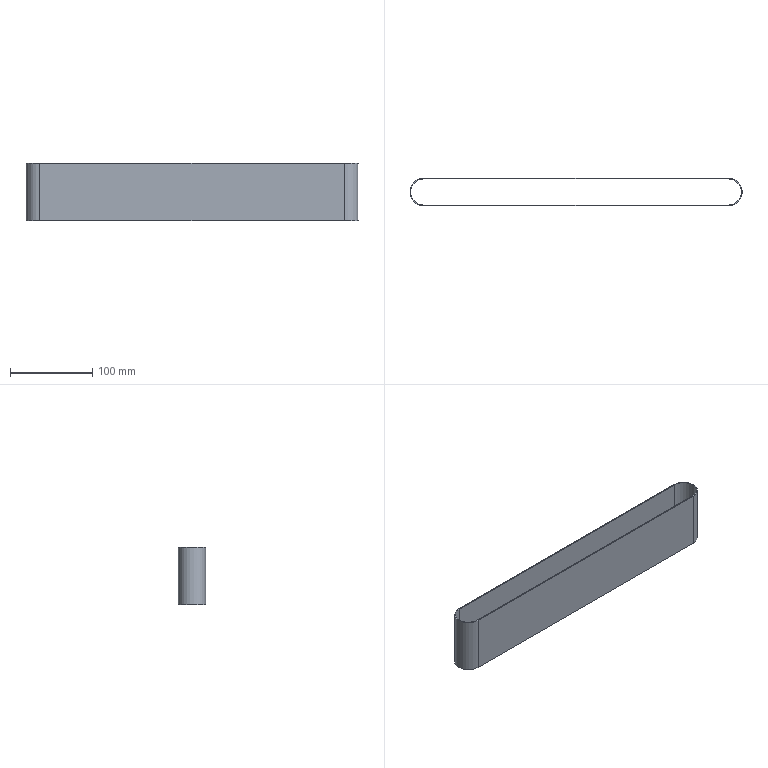Component | NX | CVSMB_70_370_H_B | 1 solid | 10 faces | box 403.8 x 33.8 x 70 mm | volume 53132 mm3 | plane 6 | cylinder 4 | commonest cylinder face diameters 33.8 x2 32 x2
STEP:
#1=CARTESIAN_POINT('',(0.,0.,0.));
#2=DIRECTION('',(0.,0.,1.));
#3=DIRECTION('',(1.,0.,0.));
#4=AXIS2_PLACEMENT_3D('',#1,#2,#3);
#5=CARTESIAN_POINT('',(-152.185,-69.989,35.5));
#6=VERTEX_POINT('',#5);
#7=CARTESIAN_POINT('',(-152.185,-36.189,35.5));
#8=VERTEX_POINT('',#7);
#9=CARTESIAN_POINT('',(-152.185,-53.089,35.5));
#10=DIRECTION('',(0.,0.,-1.));
#11=DIRECTION('',(1.,0.,0.));
#12=AXIS2_PLACEMENT_3D('',#9,#10,#11);
#13=CIRCLE('',#12,16.9);
#14=CARTESIAN_POINT('',(-152.185,-53.089,35.5));
#15=DIRECTION('',(0.,0.,-1.));
#16=DIRECTION('',(-1.,0.,0.));
#17=AXIS2_PLACEMENT_3D('',#14,#15,#16);
#18=PLANE('',#17);
#19=CARTESIAN_POINT('',(0.,0.));
#20=DIRECTION('',(-1.,0.));
#21=AXIS2_PLACEMENT_2D('',#19,#20);
#22=CIRCLE('',#21,16.9);
#23=(GEOMETRIC_REPRESENTATION_CONTEXT(2)PARAMETRIC_REPRESENTATION_CONTEXT()REPRESENTATION_CONTEXT('',''));
#24=DEFINITIONAL_REPRESENTATION('',(#22),#23);
#25=PCURVE('',#18,#24);
#26=CARTESIAN_POINT('',(-152.185,-53.089,35.5));
#27=DIRECTION('',(0.,0.,-1.));
#28=DIRECTION('',(-1.,0.,0.));
#29=AXIS2_PLACEMENT_3D('',#26,#27,#28);
#30=CYLINDRICAL_SURFACE('',#29,16.9);
#31=CARTESIAN_POINT('',(3.142,0.));
#32=DIRECTION('',(1.,0.));
#33=VECTOR('',#32,1.);
#34=LINE('',#31,#33);
#35=(GEOMETRIC_REPRESENTATION_CONTEXT(2)PARAMETRIC_REPRESENTATION_CONTEXT()REPRESENTATION_CONTEXT('',''));
#36=DEFINITIONAL_REPRESENTATION('',(#34),#35);
#37=PCURVE('',#30,#36);
#38=SURFACE_CURVE('',#13,(#25,#37),.PCURVE_S1.);
#39=EDGE_CURVE('',#6,#8,#38,.T.);
#40=ORIENTED_EDGE('',*,*,#39,.F.);
#41=CARTESIAN_POINT('',(217.815,-69.989,35.5));
#42=VERTEX_POINT('',#41);
#43=CARTESIAN_POINT('',(-152.185,-69.989,35.5));
#44=DIRECTION('',(1.,0.,0.));
#45=VECTOR('',#44,1.);
#46=LINE('',#43,#45);
#47=CARTESIAN_POINT('',(0.,-16.9));
#48=DIRECTION('',(-1.,0.));
#49=VECTOR('',#48,1.);
#50=LINE('',#47,#49);
#51=(GEOMETRIC_REPRESENTATION_CONTEXT(2)PARAMETRIC_REPRESENTATION_CONTEXT()REPRESENTATION_CONTEXT('',''));
#52=DEFINITIONAL_REPRESENTATION('',(#50),#51);
#53=PCURVE('',#18,#52);
#54=CARTESIAN_POINT('',(-152.185,-69.989,35.5));
#55=DIRECTION('',(0.,1.,0.));
#56=DIRECTION('',(0.,0.,1.));
#57=AXIS2_PLACEMENT_3D('',#54,#55,#56);
#58=PLANE('',#57);
#59=CARTESIAN_POINT('',(0.,0.));
#60=DIRECTION('',(0.,1.));
#61=VECTOR('',#60,1.);
#62=LINE('',#59,#61);
#63=(GEOMETRIC_REPRESENTATION_CONTEXT(2)PARAMETRIC_REPRESENTATION_CONTEXT()REPRESENTATION_CONTEXT('',''));
#64=DEFINITIONAL_REPRESENTATION('',(#62),#63);
#65=PCURVE('',#58,#64);
#66=SURFACE_CURVE('',#46,(#53,#65),.PCURVE_S1.);
#67=EDGE_CURVE('',#6,#42,#66,.T.);
#68=ORIENTED_EDGE('',*,*,#67,.T.);
#69=CARTESIAN_POINT('',(217.815,-36.189,35.5));
#70=VERTEX_POINT('',#69);
#71=CARTESIAN_POINT('',(217.815,-53.089,35.5));
#72=DIRECTION('',(0.,0.,-1.));
#73=DIRECTION('',(1.,0.,0.));
#74=AXIS2_PLACEMENT_3D('',#71,#72,#73);
#75=CIRCLE('',#74,16.9);
#76=CARTESIAN_POINT('',(-370.,0.));
#77=DIRECTION('',(-1.,0.));
#78=AXIS2_PLACEMENT_2D('',#76,#77);
#79=CIRCLE('',#78,16.9);
#80=(GEOMETRIC_REPRESENTATION_CONTEXT(2)PARAMETRIC_REPRESENTATION_CONTEXT()REPRESENTATION_CONTEXT('',''));
#81=DEFINITIONAL_REPRESENTATION('',(#79),#80);
#82=PCURVE('',#18,#81);
#83=CARTESIAN_POINT('',(217.815,-53.089,35.5));
#84=DIRECTION('',(0.,0.,-1.));
#85=DIRECTION('',(-1.,0.,0.));
#86=AXIS2_PLACEMENT_3D('',#83,#84,#85);
#87=CYLINDRICAL_SURFACE('',#86,16.9);
#88=CARTESIAN_POINT('',(-3.142,0.));
#89=DIRECTION('',(1.,0.));
#90=VECTOR('',#89,1.);
#91=LINE('',#88,#90);
#92=(GEOMETRIC_REPRESENTATION_CONTEXT(2)PARAMETRIC_REPRESENTATION_CONTEXT()REPRESENTATION_CONTEXT('',''));
#93=DEFINITIONAL_REPRESENTATION('',(#91),#92);
#94=PCURVE('',#87,#93);
#95=SURFACE_CURVE('',#75,(#82,#94),.PCURVE_S1.);
#96=EDGE_CURVE('',#70,#42,#95,.T.);
#97=ORIENTED_EDGE('',*,*,#96,.F.);
#98=CARTESIAN_POINT('',(217.815,-36.189,35.5));
#99=DIRECTION('',(-1.,0.,0.));
#100=VECTOR('',#99,1.);
#101=LINE('',#98,#100);
#102=CARTESIAN_POINT('',(-370.,16.9));
#103=DIRECTION('',(1.,0.));
#104=VECTOR('',#103,1.);
#105=LINE('',#102,#104);
#106=(GEOMETRIC_REPRESENTATION_CONTEXT(2)PARAMETRIC_REPRESENTATION_CONTEXT()REPRESENTATION_CONTEXT('',''));
#107=DEFINITIONAL_REPRESENTATION('',(#105),#106);
#108=PCURVE('',#18,#107);
#109=CARTESIAN_POINT('',(217.815,-36.189,35.5));
#110=DIRECTION('',(0.,-1.,0.));
#111=DIRECTION('',(0.,0.,-1.));
#112=AXIS2_PLACEMENT_3D('',#109,#110,#111);
#113=PLANE('',#112);
#114=CARTESIAN_POINT('',(0.,0.));
#115=DIRECTION('',(0.,-1.));
#116=VECTOR('',#115,1.);
#117=LINE('',#114,#116);
#118=(GEOMETRIC_REPRESENTATION_CONTEXT(2)PARAMETRIC_REPRESENTATION_CONTEXT()REPRESENTATION_CONTEXT('',''));
#119=DEFINITIONAL_REPRESENTATION('',(#117),#118);
#120=PCURVE('',#113,#119);
#121=SURFACE_CURVE('',#101,(#108,#120),.PCURVE_S1.);
#122=EDGE_CURVE('',#70,#8,#121,.T.);
#123=ORIENTED_EDGE('',*,*,#122,.T.);
#124=EDGE_LOOP('',(#40,#68,#97,#123));
#125=FACE_BOUND('',#124,.T.);
#126=CARTESIAN_POINT('',(-152.185,-69.089,35.5));
#127=VERTEX_POINT('',#126);
#128=CARTESIAN_POINT('',(217.815,-69.089,35.5));
#129=VERTEX_POINT('',#128);
#130=CARTESIAN_POINT('',(-152.185,-69.089,35.5));
#131=DIRECTION('',(1.,0.,0.));
#132=VECTOR('',#131,1.);
#133=LINE('',#130,#132);
#134=CARTESIAN_POINT('',(0.,-16.));
#135=DIRECTION('',(-1.,0.));
#136=VECTOR('',#135,1.);
#137=LINE('',#134,#136);
#138=(GEOMETRIC_REPRESENTATION_CONTEXT(2)PARAMETRIC_REPRESENTATION_CONTEXT()REPRESENTATION_CONTEXT('',''));
#139=DEFINITIONAL_REPRESENTATION('',(#137),#138);
#140=PCURVE('',#18,#139);
#141=CARTESIAN_POINT('',(-152.185,-69.089,35.5));
#142=DIRECTION('',(0.,1.,0.));
#143=DIRECTION('',(0.,0.,1.));
#144=AXIS2_PLACEMENT_3D('',#141,#142,#143);
#145=PLANE('',#144);
#146=CARTESIAN_POINT('',(0.,0.));
#147=DIRECTION('',(0.,1.));
#148=VECTOR('',#147,1.);
#149=LINE('',#146,#148);
#150=(GEOMETRIC_REPRESENTATION_CONTEXT(2)PARAMETRIC_REPRESENTATION_CONTEXT()REPRESENTATION_CONTEXT('',''));
#151=DEFINITIONAL_REPRESENTATION('',(#149),#150);
#152=PCURVE('',#145,#151);
#153=SURFACE_CURVE('',#133,(#140,#152),.PCURVE_S1.);
#154=EDGE_CURVE('',#127,#129,#153,.T.);
#155=ORIENTED_EDGE('',*,*,#154,.F.);
#156=CARTESIAN_POINT('',(-152.185,-37.089,35.5));
#157=VERTEX_POINT('',#156);
#158=CARTESIAN_POINT('',(-152.185,-53.089,35.5));
#159=DIRECTION('',(0.,0.,-1.));
#160=DIRECTION('',(1.,0.,0.));
#161=AXIS2_PLACEMENT_3D('',#158,#159,#160);
#162=CIRCLE('',#161,16.);
#163=CARTESIAN_POINT('',(0.,0.));
#164=DIRECTION('',(-1.,0.));
#165=AXIS2_PLACEMENT_2D('',#163,#164);
#166=CIRCLE('',#165,16.);
#167=(GEOMETRIC_REPRESENTATION_CONTEXT(2)PARAMETRIC_REPRESENTATION_CONTEXT()REPRESENTATION_CONTEXT('',''));
#168=DEFINITIONAL_REPRESENTATION('',(#166),#167);
#169=PCURVE('',#18,#168);
#170=CARTESIAN_POINT('',(-152.185,-53.089,35.5));
#171=DIRECTION('',(0.,0.,-1.));
#172=DIRECTION('',(-1.,0.,0.));
#173=AXIS2_PLACEMENT_3D('',#170,#171,#172);
#174=CYLINDRICAL_SURFACE('',#173,16.);
#175=CARTESIAN_POINT('',(3.142,0.));
#176=DIRECTION('',(1.,0.));
#177=VECTOR('',#176,1.);
#178=LINE('',#175,#177);
#179=(GEOMETRIC_REPRESENTATION_CONTEXT(2)PARAMETRIC_REPRESENTATION_CONTEXT()REPRESENTATION_CONTEXT('',''));
#180=DEFINITIONAL_REPRESENTATION('',(#178),#179);
#181=PCURVE('',#174,#180);
#182=SURFACE_CURVE('',#162,(#169,#181),.PCURVE_S1.);
#183=EDGE_CURVE('',#127,#157,#182,.T.);
#184=ORIENTED_EDGE('',*,*,#183,.T.);
#185=CARTESIAN_POINT('',(217.815,-37.089,35.5));
#186=VERTEX_POINT('',#185);
#187=CARTESIAN_POINT('',(217.815,-37.089,35.5));
#188=DIRECTION('',(-1.,0.,0.));
#189=VECTOR('',#188,1.);
#190=LINE('',#187,#189);
#191=CARTESIAN_POINT('',(-370.,16.));
#192=DIRECTION('',(1.,0.));
#193=VECTOR('',#192,1.);
#194=LINE('',#191,#193);
#195=(GEOMETRIC_REPRESENTATION_CONTEXT(2)PARAMETRIC_REPRESENTATION_CONTEXT()REPRESENTATION_CONTEXT('',''));
#196=DEFINITIONAL_REPRESENTATION('',(#194),#195);
#197=PCURVE('',#18,#196);
#198=CARTESIAN_POINT('',(217.815,-37.089,35.5));
#199=DIRECTION('',(0.,-1.,0.));
#200=DIRECTION('',(0.,0.,-1.));
#201=AXIS2_PLACEMENT_3D('',#198,#199,#200);
#202=PLANE('',#201);
#203=CARTESIAN_POINT('',(0.,0.));
#204=DIRECTION('',(0.,-1.));
#205=VECTOR('',#204,1.);
#206=LINE('',#203,#205);
#207=(GEOMETRIC_REPRESENTATION_CONTEXT(2)PARAMETRIC_REPRESENTATION_CONTEXT()REPRESENTATION_CONTEXT('',''));
#208=DEFINITIONAL_REPRESENTATION('',(#206),#207);
#209=PCURVE('',#202,#208);
#210=SURFACE_CURVE('',#190,(#197,#209),.PCURVE_S1.);
#211=EDGE_CURVE('',#186,#157,#210,.T.);
#212=ORIENTED_EDGE('',*,*,#211,.F.);
#213=CARTESIAN_POINT('',(217.815,-53.089,35.5));
#214=DIRECTION('',(0.,0.,-1.));
#215=DIRECTION('',(1.,0.,0.));
#216=AXIS2_PLACEMENT_3D('',#213,#214,#215);
#217=CIRCLE('',#216,16.);
#218=CARTESIAN_POINT('',(-370.,0.));
#219=DIRECTION('',(-1.,0.));
#220=AXIS2_PLACEMENT_2D('',#218,#219);
#221=CIRCLE('',#220,16.);
#222=(GEOMETRIC_REPRESENTATION_CONTEXT(2)PARAMETRIC_REPRESENTATION_CONTEXT()REPRESENTATION_CONTEXT('',''));
#223=DEFINITIONAL_REPRESENTATION('',(#221),#222);
#224=PCURVE('',#18,#223);
#225=CARTESIAN_POINT('',(217.815,-53.089,35.5));
#226=DIRECTION('',(0.,0.,-1.));
#227=DIRECTION('',(-1.,0.,0.));
#228=AXIS2_PLACEMENT_3D('',#225,#226,#227);
#229=CYLINDRICAL_SURFACE('',#228,16.);
#230=CARTESIAN_POINT('',(-3.142,0.));
#231=DIRECTION('',(1.,0.));
#232=VECTOR('',#231,1.);
#233=LINE('',#230,#232);
#234=(GEOMETRIC_REPRESENTATION_CONTEXT(2)PARAMETRIC_REPRESENTATION_CONTEXT()REPRESENTATION_CONTEXT('',''));
#235=DEFINITIONAL_REPRESENTATION('',(#233),#234);
#236=PCURVE('',#229,#235);
#237=SURFACE_CURVE('',#217,(#224,#236),.PCURVE_S1.);
#238=EDGE_CURVE('',#186,#129,#237,.T.);
#239=ORIENTED_EDGE('',*,*,#238,.T.);
#240=EDGE_LOOP('',(#155,#184,#212,#239));
#241=FACE_BOUND('',#240,.T.);
#242=ADVANCED_FACE('',(#125,#241),#18,.F.);
#243=CARTESIAN_POINT('',(-152.185,-69.989,-34.5));
#244=VERTEX_POINT('',#243);
#245=CARTESIAN_POINT('',(-152.185,-36.189,-34.5));
#246=VERTEX_POINT('',#245);
#247=CARTESIAN_POINT('',(-152.185,-53.089,-34.5));
#248=DIRECTION('',(0.,0.,-1.));
#249=DIRECTION('',(1.,0.,0.));
#250=AXIS2_PLACEMENT_3D('',#247,#248,#249);
#251=CIRCLE('',#250,16.9);
#252=CARTESIAN_POINT('',(-152.185,-53.089,-34.5));
#253=DIRECTION('',(0.,0.,-1.));
#254=DIRECTION('',(-1.,0.,0.));
#255=AXIS2_PLACEMENT_3D('',#252,#253,#254);
#256=PLANE('',#255);
#257=CARTESIAN_POINT('',(0.,0.));
#258=DIRECTION('',(-1.,0.));
#259=AXIS2_PLACEMENT_2D('',#257,#258);
#260=CIRCLE('',#259,16.9);
#261=(GEOMETRIC_REPRESENTATION_CONTEXT(2)PARAMETRIC_REPRESENTATION_CONTEXT()REPRESENTATION_CONTEXT('',''));
#262=DEFINITIONAL_REPRESENTATION('',(#260),#261);
#263=PCURVE('',#256,#262);
#264=CARTESIAN_POINT('',(3.142,70.));
#265=DIRECTION('',(1.,0.));
#266=VECTOR('',#265,1.);
#267=LINE('',#264,#266);
#268=(GEOMETRIC_REPRESENTATION_CONTEXT(2)PARAMETRIC_REPRESENTATION_CONTEXT()REPRESENTATION_CONTEXT('',''));
#269=DEFINITIONAL_REPRESENTATION('',(#267),#268);
#270=PCURVE('',#30,#269);
#271=SURFACE_CURVE('',#251,(#263,#270),.PCURVE_S1.);
#272=EDGE_CURVE('',#244,#246,#271,.T.);
#273=ORIENTED_EDGE('',*,*,#272,.T.);
#274=CARTESIAN_POINT('',(217.815,-36.189,-34.5));
#275=VERTEX_POINT('',#274);
#276=CARTESIAN_POINT('',(217.815,-36.189,-34.5));
#277=DIRECTION('',(-1.,0.,0.));
#278=VECTOR('',#277,1.);
#279=LINE('',#276,#278);
#280=CARTESIAN_POINT('',(-370.,16.9));
#281=DIRECTION('',(1.,0.));
#282=VECTOR('',#281,1.);
#283=LINE('',#280,#282);
#284=(GEOMETRIC_REPRESENTATION_CONTEXT(2)PARAMETRIC_REPRESENTATION_CONTEXT()REPRESENTATION_CONTEXT('',''));
#285=DEFINITIONAL_REPRESENTATION('',(#283),#284);
#286=PCURVE('',#256,#285);
#287=CARTESIAN_POINT('',(70.,0.));
#288=DIRECTION('',(0.,-1.));
#289=VECTOR('',#288,1.);
#290=LINE('',#287,#289);
#291=(GEOMETRIC_REPRESENTATION_CONTEXT(2)PARAMETRIC_REPRESENTATION_CONTEXT()REPRESENTATION_CONTEXT('',''));
#292=DEFINITIONAL_REPRESENTATION('',(#290),#291);
#293=PCURVE('',#113,#292);
#294=SURFACE_CURVE('',#279,(#286,#293),.PCURVE_S1.);
#295=EDGE_CURVE('',#275,#246,#294,.T.);
#296=ORIENTED_EDGE('',*,*,#295,.F.);
#297=CARTESIAN_POINT('',(217.815,-69.989,-34.5));
#298=VERTEX_POINT('',#297);
#299=CARTESIAN_POINT('',(217.815,-53.089,-34.5));
#300=DIRECTION('',(0.,0.,-1.));
#301=DIRECTION('',(1.,0.,0.));
#302=AXIS2_PLACEMENT_3D('',#299,#300,#301);
#303=CIRCLE('',#302,16.9);
#304=CARTESIAN_POINT('',(-370.,0.));
#305=DIRECTION('',(-1.,0.));
#306=AXIS2_PLACEMENT_2D('',#304,#305);
#307=CIRCLE('',#306,16.9);
#308=(GEOMETRIC_REPRESENTATION_CONTEXT(2)PARAMETRIC_REPRESENTATION_CONTEXT()REPRESENTATION_CONTEXT('',''));
#309=DEFINITIONAL_REPRESENTATION('',(#307),#308);
#310=PCURVE('',#256,#309);
#311=CARTESIAN_POINT('',(-3.142,70.));
#312=DIRECTION('',(1.,0.));
#313=VECTOR('',#312,1.);
#314=LINE('',#311,#313);
#315=(GEOMETRIC_REPRESENTATION_CONTEXT(2)PARAMETRIC_REPRESENTATION_CONTEXT()REPRESENTATION_CONTEXT('',''));
#316=DEFINITIONAL_REPRESENTATION('',(#314),#315);
#317=PCURVE('',#87,#316);
#318=SURFACE_CURVE('',#303,(#310,#317),.PCURVE_S1.);
#319=EDGE_CURVE('',#275,#298,#318,.T.);
#320=ORIENTED_EDGE('',*,*,#319,.T.);
#321=CARTESIAN_POINT('',(-152.185,-69.989,-34.5));
#322=DIRECTION('',(1.,0.,0.));
#323=VECTOR('',#322,1.);
#324=LINE('',#321,#323);
#325=CARTESIAN_POINT('',(0.,-16.9));
#326=DIRECTION('',(-1.,0.));
#327=VECTOR('',#326,1.);
#328=LINE('',#325,#327);
#329=(GEOMETRIC_REPRESENTATION_CONTEXT(2)PARAMETRIC_REPRESENTATION_CONTEXT()REPRESENTATION_CONTEXT('',''));
#330=DEFINITIONAL_REPRESENTATION('',(#328),#329);
#331=PCURVE('',#256,#330);
#332=CARTESIAN_POINT('',(-70.,0.));
#333=DIRECTION('',(0.,1.));
#334=VECTOR('',#333,1.);
#335=LINE('',#332,#334);
#336=(GEOMETRIC_REPRESENTATION_CONTEXT(2)PARAMETRIC_REPRESENTATION_CONTEXT()REPRESENTATION_CONTEXT('',''));
#337=DEFINITIONAL_REPRESENTATION('',(#335),#336);
#338=PCURVE('',#58,#337);
#339=SURFACE_CURVE('',#324,(#331,#338),.PCURVE_S1.);
#340=EDGE_CURVE('',#244,#298,#339,.T.);
#341=ORIENTED_EDGE('',*,*,#340,.F.);
#342=EDGE_LOOP('',(#273,#296,#320,#341));
#343=FACE_BOUND('',#342,.T.);
#344=CARTESIAN_POINT('',(-152.185,-69.089,-34.5));
#345=VERTEX_POINT('',#344);
#346=CARTESIAN_POINT('',(-152.185,-37.089,-34.5));
#347=VERTEX_POINT('',#346);
#348=CARTESIAN_POINT('',(-152.185,-53.089,-34.5));
#349=DIRECTION('',(0.,0.,-1.));
#350=DIRECTION('',(1.,0.,0.));
#351=AXIS2_PLACEMENT_3D('',#348,#349,#350);
#352=CIRCLE('',#351,16.);
#353=CARTESIAN_POINT('',(0.,0.));
#354=DIRECTION('',(-1.,0.));
#355=AXIS2_PLACEMENT_2D('',#353,#354);
#356=CIRCLE('',#355,16.);
#357=(GEOMETRIC_REPRESENTATION_CONTEXT(2)PARAMETRIC_REPRESENTATION_CONTEXT()REPRESENTATION_CONTEXT('',''));
#358=DEFINITIONAL_REPRESENTATION('',(#356),#357);
#359=PCURVE('',#256,#358);
#360=CARTESIAN_POINT('',(3.142,70.));
#361=DIRECTION('',(1.,0.));
#362=VECTOR('',#361,1.);
#363=LINE('',#360,#362);
#364=(GEOMETRIC_REPRESENTATION_CONTEXT(2)PARAMETRIC_REPRESENTATION_CONTEXT()REPRESENTATION_CONTEXT('',''));
#365=DEFINITIONAL_REPRESENTATION('',(#363),#364);
#366=PCURVE('',#174,#365);
#367=SURFACE_CURVE('',#352,(#359,#366),.PCURVE_S1.);
#368=EDGE_CURVE('',#345,#347,#367,.T.);
#369=ORIENTED_EDGE('',*,*,#368,.F.);
#370=CARTESIAN_POINT('',(217.815,-69.089,-34.5));
#371=VERTEX_POINT('',#370);
#372=CARTESIAN_POINT('',(-152.185,-69.089,-34.5));
#373=DIRECTION('',(1.,0.,0.));
#374=VECTOR('',#373,1.);
#375=LINE('',#372,#374);
#376=CARTESIAN_POINT('',(0.,-16.));
#377=DIRECTION('',(-1.,0.));
#378=VECTOR('',#377,1.);
#379=LINE('',#376,#378);
#380=(GEOMETRIC_REPRESENTATION_CONTEXT(2)PARAMETRIC_REPRESENTATION_CONTEXT()REPRESENTATION_CONTEXT('',''));
#381=DEFINITIONAL_REPRESENTATION('',(#379),#380);
#382=PCURVE('',#256,#381);
#383=CARTESIAN_POINT('',(-70.,0.));
#384=DIRECTION('',(0.,1.));
#385=VECTOR('',#384,1.);
#386=LINE('',#383,#385);
#387=(GEOMETRIC_REPRESENTATION_CONTEXT(2)PARAMETRIC_REPRESENTATION_CONTEXT()REPRESENTATION_CONTEXT('',''));
#388=DEFINITIONAL_REPRESENTATION('',(#386),#387);
#389=PCURVE('',#145,#388);
#390=SURFACE_CURVE('',#375,(#382,#389),.PCURVE_S1.);
#391=EDGE_CURVE('',#345,#371,#390,.T.);
#392=ORIENTED_EDGE('',*,*,#391,.T.);
#393=CARTESIAN_POINT('',(217.815,-37.089,-34.5));
#394=VERTEX_POINT('',#393);
#395=CARTESIAN_POINT('',(217.815,-53.089,-34.5));
#396=DIRECTION('',(0.,0.,-1.));
#397=DIRECTION('',(1.,0.,0.));
#398=AXIS2_PLACEMENT_3D('',#395,#396,#397);
#399=CIRCLE('',#398,16.);
#400=CARTESIAN_POINT('',(-370.,0.));
#401=DIRECTION('',(-1.,0.));
#402=AXIS2_PLACEMENT_2D('',#400,#401);
#403=CIRCLE('',#402,16.);
#404=(GEOMETRIC_REPRESENTATION_CONTEXT(2)PARAMETRIC_REPRESENTATION_CONTEXT()REPRESENTATION_CONTEXT('',''));
#405=DEFINITIONAL_REPRESENTATION('',(#403),#404);
#406=PCURVE('',#256,#405);
#407=CARTESIAN_POINT('',(-3.142,70.));
#408=DIRECTION('',(1.,0.));
#409=VECTOR('',#408,1.);
#410=LINE('',#407,#409);
#411=(GEOMETRIC_REPRESENTATION_CONTEXT(2)PARAMETRIC_REPRESENTATION_CONTEXT()REPRESENTATION_CONTEXT('',''));
#412=DEFINITIONAL_REPRESENTATION('',(#410),#411);
#413=PCURVE('',#229,#412);
#414=SURFACE_CURVE('',#399,(#406,#413),.PCURVE_S1.);
#415=EDGE_CURVE('',#394,#371,#414,.T.);
#416=ORIENTED_EDGE('',*,*,#415,.F.);
#417=CARTESIAN_POINT('',(217.815,-37.089,-34.5));
#418=DIRECTION('',(-1.,0.,0.));
#419=VECTOR('',#418,1.);
#420=LINE('',#417,#419);
#421=CARTESIAN_POINT('',(-370.,16.));
#422=DIRECTION('',(1.,0.));
#423=VECTOR('',#422,1.);
#424=LINE('',#421,#423);
#425=(GEOMETRIC_REPRESENTATION_CONTEXT(2)PARAMETRIC_REPRESENTATION_CONTEXT()REPRESENTATION_CONTEXT('',''));
#426=DEFINITIONAL_REPRESENTATION('',(#424),#425);
#427=PCURVE('',#256,#426);
#428=CARTESIAN_POINT('',(70.,0.));
#429=DIRECTION('',(0.,-1.));
#430=VECTOR('',#429,1.);
#431=LINE('',#428,#430);
#432=(GEOMETRIC_REPRESENTATION_CONTEXT(2)PARAMETRIC_REPRESENTATION_CONTEXT()REPRESENTATION_CONTEXT('',''));
#433=DEFINITIONAL_REPRESENTATION('',(#431),#432);
#434=PCURVE('',#202,#433);
#435=SURFACE_CURVE('',#420,(#427,#434),.PCURVE_S1.);
#436=EDGE_CURVE('',#394,#347,#435,.T.);
#437=ORIENTED_EDGE('',*,*,#436,.T.);
#438=EDGE_LOOP('',(#369,#392,#416,#437));
#439=FACE_BOUND('',#438,.T.);
#440=ADVANCED_FACE('',(#343,#439),#256,.T.);
#441=ORIENTED_EDGE('',*,*,#272,.F.);
#442=CARTESIAN_POINT('',(-152.185,-69.989,35.5));
#443=DIRECTION('',(0.,0.,-1.));
#444=VECTOR('',#443,1.);
#445=LINE('',#442,#444);
#446=CARTESIAN_POINT('',(4.712,0.));
#447=DIRECTION('',(0.,1.));
#448=VECTOR('',#447,1.);
#449=LINE('',#446,#448);
#450=(GEOMETRIC_REPRESENTATION_CONTEXT(2)PARAMETRIC_REPRESENTATION_CONTEXT()REPRESENTATION_CONTEXT('',''));
#451=DEFINITIONAL_REPRESENTATION('',(#449),#450);
#452=PCURVE('',#30,#451);
#453=CARTESIAN_POINT('',(0.,0.));
#454=DIRECTION('',(-1.,0.));
#455=VECTOR('',#454,1.);
#456=LINE('',#453,#455);
#457=(GEOMETRIC_REPRESENTATION_CONTEXT(2)PARAMETRIC_REPRESENTATION_CONTEXT()REPRESENTATION_CONTEXT('',''));
#458=DEFINITIONAL_REPRESENTATION('',(#456),#457);
#459=PCURVE('',#58,#458);
#460=SURFACE_CURVE('',#445,(#452,#459),.PCURVE_S1.);
#461=EDGE_CURVE('',#6,#244,#460,.T.);
#462=ORIENTED_EDGE('',*,*,#461,.F.);
#463=ORIENTED_EDGE('',*,*,#39,.T.);
#464=CARTESIAN_POINT('',(-152.185,-36.189,35.5));
#465=DIRECTION('',(0.,0.,-1.));
#466=VECTOR('',#465,1.);
#467=LINE('',#464,#466);
#468=CARTESIAN_POINT('',(7.854,0.));
#469=DIRECTION('',(0.,1.));
#470=VECTOR('',#469,1.);
#471=LINE('',#468,#470);
#472=(GEOMETRIC_REPRESENTATION_CONTEXT(2)PARAMETRIC_REPRESENTATION_CONTEXT()REPRESENTATION_CONTEXT('',''));
#473=DEFINITIONAL_REPRESENTATION('',(#471),#472);
#474=PCURVE('',#30,#473);
#475=CARTESIAN_POINT('',(0.,-370.));
#476=DIRECTION('',(1.,0.));
#477=VECTOR('',#476,1.);
#478=LINE('',#475,#477);
#479=(GEOMETRIC_REPRESENTATION_CONTEXT(2)PARAMETRIC_REPRESENTATION_CONTEXT()REPRESENTATION_CONTEXT('',''));
#480=DEFINITIONAL_REPRESENTATION('',(#478),#479);
#481=PCURVE('',#113,#480);
#482=SURFACE_CURVE('',#467,(#474,#481),.PCURVE_S1.);
#483=EDGE_CURVE('',#8,#246,#482,.T.);
#484=ORIENTED_EDGE('',*,*,#483,.T.);
#485=EDGE_LOOP('',(#441,#462,#463,#484));
#486=FACE_BOUND('',#485,.T.);
#487=ADVANCED_FACE('',(#486),#30,.T.);
#488=ORIENTED_EDGE('',*,*,#295,.T.);
#489=ORIENTED_EDGE('',*,*,#483,.F.);
#490=ORIENTED_EDGE('',*,*,#122,.F.);
#491=CARTESIAN_POINT('',(217.815,-36.189,35.5));
#492=DIRECTION('',(0.,0.,-1.));
#493=VECTOR('',#492,1.);
#494=LINE('',#491,#493);
#495=CARTESIAN_POINT('',(0.,0.));
#496=DIRECTION('',(1.,0.));
#497=VECTOR('',#496,1.);
#498=LINE('',#495,#497);
#499=(GEOMETRIC_REPRESENTATION_CONTEXT(2)PARAMETRIC_REPRESENTATION_CONTEXT()REPRESENTATION_CONTEXT('',''));
#500=DEFINITIONAL_REPRESENTATION('',(#498),#499);
#501=PCURVE('',#113,#500);
#502=CARTESIAN_POINT('',(1.571,0.));
#503=DIRECTION('',(0.,1.));
#504=VECTOR('',#503,1.);
#505=LINE('',#502,#504);
#506=(GEOMETRIC_REPRESENTATION_CONTEXT(2)PARAMETRIC_REPRESENTATION_CONTEXT()REPRESENTATION_CONTEXT('',''));
#507=DEFINITIONAL_REPRESENTATION('',(#505),#506);
#508=PCURVE('',#87,#507);
#509=SURFACE_CURVE('',#494,(#501,#508),.PCURVE_S1.);
#510=EDGE_CURVE('',#70,#275,#509,.T.);
#511=ORIENTED_EDGE('',*,*,#510,.T.);
#512=EDGE_LOOP('',(#488,#489,#490,#511));
#513=FACE_BOUND('',#512,.T.);
#514=ADVANCED_FACE('',(#513),#113,.F.);
#515=ORIENTED_EDGE('',*,*,#319,.F.);
#516=ORIENTED_EDGE('',*,*,#510,.F.);
#517=ORIENTED_EDGE('',*,*,#96,.T.);
#518=CARTESIAN_POINT('',(217.815,-69.989,35.5));
#519=DIRECTION('',(0.,0.,-1.));
#520=VECTOR('',#519,1.);
#521=LINE('',#518,#520);
#522=CARTESIAN_POINT('',(4.712,0.));
#523=DIRECTION('',(0.,1.));
#524=VECTOR('',#523,1.);
#525=LINE('',#522,#524);
#526=(GEOMETRIC_REPRESENTATION_CONTEXT(2)PARAMETRIC_REPRESENTATION_CONTEXT()REPRESENTATION_CONTEXT('',''));
#527=DEFINITIONAL_REPRESENTATION('',(#525),#526);
#528=PCURVE('',#87,#527);
#529=CARTESIAN_POINT('',(0.,370.));
#530=DIRECTION('',(-1.,0.));
#531=VECTOR('',#530,1.);
#532=LINE('',#529,#531);
#533=(GEOMETRIC_REPRESENTATION_CONTEXT(2)PARAMETRIC_REPRESENTATION_CONTEXT()REPRESENTATION_CONTEXT('',''));
#534=DEFINITIONAL_REPRESENTATION('',(#532),#533);
#535=PCURVE('',#58,#534);
#536=SURFACE_CURVE('',#521,(#528,#535),.PCURVE_S1.);
#537=EDGE_CURVE('',#42,#298,#536,.T.);
#538=ORIENTED_EDGE('',*,*,#537,.T.);
#539=EDGE_LOOP('',(#515,#516,#517,#538));
#540=FACE_BOUND('',#539,.T.);
#541=ADVANCED_FACE('',(#540),#87,.T.);
#542=ORIENTED_EDGE('',*,*,#340,.T.);
#543=ORIENTED_EDGE('',*,*,#537,.F.);
#544=ORIENTED_EDGE('',*,*,#67,.F.);
#545=ORIENTED_EDGE('',*,*,#461,.T.);
#546=EDGE_LOOP('',(#542,#543,#544,#545));
#547=FACE_BOUND('',#546,.T.);
#548=ADVANCED_FACE('',(#547),#58,.F.);
#549=ORIENTED_EDGE('',*,*,#391,.F.);
#550=CARTESIAN_POINT('',(-152.185,-69.089,35.5));
#551=DIRECTION('',(0.,0.,-1.));
#552=VECTOR('',#551,1.);
#553=LINE('',#550,#552);
#554=CARTESIAN_POINT('',(0.,0.));
#555=DIRECTION('',(-1.,0.));
#556=VECTOR('',#555,1.);
#557=LINE('',#554,#556);
#558=(GEOMETRIC_REPRESENTATION_CONTEXT(2)PARAMETRIC_REPRESENTATION_CONTEXT()REPRESENTATION_CONTEXT('',''));
#559=DEFINITIONAL_REPRESENTATION('',(#557),#558);
#560=PCURVE('',#145,#559);
#561=CARTESIAN_POINT('',(4.712,0.));
#562=DIRECTION('',(0.,1.));
#563=VECTOR('',#562,1.);
#564=LINE('',#561,#563);
#565=(GEOMETRIC_REPRESENTATION_CONTEXT(2)PARAMETRIC_REPRESENTATION_CONTEXT()REPRESENTATION_CONTEXT('',''));
#566=DEFINITIONAL_REPRESENTATION('',(#564),#565);
#567=PCURVE('',#174,#566);
#568=SURFACE_CURVE('',#553,(#560,#567),.PCURVE_S1.);
#569=EDGE_CURVE('',#127,#345,#568,.T.);
#570=ORIENTED_EDGE('',*,*,#569,.F.);
#571=ORIENTED_EDGE('',*,*,#154,.T.);
#572=CARTESIAN_POINT('',(217.815,-69.089,35.5));
#573=DIRECTION('',(0.,0.,-1.));
#574=VECTOR('',#573,1.);
#575=LINE('',#572,#574);
#576=CARTESIAN_POINT('',(0.,370.));
#577=DIRECTION('',(-1.,0.));
#578=VECTOR('',#577,1.);
#579=LINE('',#576,#578);
#580=(GEOMETRIC_REPRESENTATION_CONTEXT(2)PARAMETRIC_REPRESENTATION_CONTEXT()REPRESENTATION_CONTEXT('',''));
#581=DEFINITIONAL_REPRESENTATION('',(#579),#580);
#582=PCURVE('',#145,#581);
#583=CARTESIAN_POINT('',(4.712,0.));
#584=DIRECTION('',(0.,1.));
#585=VECTOR('',#584,1.);
#586=LINE('',#583,#585);
#587=(GEOMETRIC_REPRESENTATION_CONTEXT(2)PARAMETRIC_REPRESENTATION_CONTEXT()REPRESENTATION_CONTEXT('',''));
#588=DEFINITIONAL_REPRESENTATION('',(#586),#587);
#589=PCURVE('',#229,#588);
#590=SURFACE_CURVE('',#575,(#582,#589),.PCURVE_S1.);
#591=EDGE_CURVE('',#129,#371,#590,.T.);
#592=ORIENTED_EDGE('',*,*,#591,.T.);
#593=EDGE_LOOP('',(#549,#570,#571,#592));
#594=FACE_BOUND('',#593,.T.);
#595=ADVANCED_FACE('',(#594),#145,.T.);
#596=CARTESIAN_POINT('',(217.815,-37.089,35.5));
#597=DIRECTION('',(0.,0.,-1.));
#598=VECTOR('',#597,1.);
#599=LINE('',#596,#598);
#600=CARTESIAN_POINT('',(1.571,0.));
#601=DIRECTION('',(0.,1.));
#602=VECTOR('',#601,1.);
#603=LINE('',#600,#602);
#604=(GEOMETRIC_REPRESENTATION_CONTEXT(2)PARAMETRIC_REPRESENTATION_CONTEXT()REPRESENTATION_CONTEXT('',''));
#605=DEFINITIONAL_REPRESENTATION('',(#603),#604);
#606=PCURVE('',#229,#605);
#607=CARTESIAN_POINT('',(0.,0.));
#608=DIRECTION('',(1.,0.));
#609=VECTOR('',#608,1.);
#610=LINE('',#607,#609);
#611=(GEOMETRIC_REPRESENTATION_CONTEXT(2)PARAMETRIC_REPRESENTATION_CONTEXT()REPRESENTATION_CONTEXT('',''));
#612=DEFINITIONAL_REPRESENTATION('',(#610),#611);
#613=PCURVE('',#202,#612);
#614=SURFACE_CURVE('',#599,(#606,#613),.PCURVE_S1.);
#615=EDGE_CURVE('',#186,#394,#614,.T.);
#616=ORIENTED_EDGE('',*,*,#615,.F.);
#617=ORIENTED_EDGE('',*,*,#238,.T.);
#618=ORIENTED_EDGE('',*,*,#591,.T.);
#619=ORIENTED_EDGE('',*,*,#415,.F.);
#620=EDGE_LOOP('',(#616,#617,#618,#619));
#621=FACE_BOUND('',#620,.F.);
#622=ADVANCED_FACE('',(#621),#229,.F.);
#623=ORIENTED_EDGE('',*,*,#436,.F.);
#624=ORIENTED_EDGE('',*,*,#615,.F.);
#625=ORIENTED_EDGE('',*,*,#211,.T.);
#626=CARTESIAN_POINT('',(-152.185,-37.089,35.5));
#627=DIRECTION('',(0.,0.,-1.));
#628=VECTOR('',#627,1.);
#629=LINE('',#626,#628);
#630=CARTESIAN_POINT('',(0.,-370.));
#631=DIRECTION('',(1.,0.));
#632=VECTOR('',#631,1.);
#633=LINE('',#630,#632);
#634=(GEOMETRIC_REPRESENTATION_CONTEXT(2)PARAMETRIC_REPRESENTATION_CONTEXT()REPRESENTATION_CONTEXT('',''));
#635=DEFINITIONAL_REPRESENTATION('',(#633),#634);
#636=PCURVE('',#202,#635);
#637=CARTESIAN_POINT('',(7.854,0.));
#638=DIRECTION('',(0.,1.));
#639=VECTOR('',#638,1.);
#640=LINE('',#637,#639);
#641=(GEOMETRIC_REPRESENTATION_CONTEXT(2)PARAMETRIC_REPRESENTATION_CONTEXT()REPRESENTATION_CONTEXT('',''));
#642=DEFINITIONAL_REPRESENTATION('',(#640),#641);
#643=PCURVE('',#174,#642);
#644=SURFACE_CURVE('',#629,(#636,#643),.PCURVE_S1.);
#645=EDGE_CURVE('',#157,#347,#644,.T.);
#646=ORIENTED_EDGE('',*,*,#645,.T.);
#647=EDGE_LOOP('',(#623,#624,#625,#646));
#648=FACE_BOUND('',#647,.T.);
#649=ADVANCED_FACE('',(#648),#202,.T.);
#650=ORIENTED_EDGE('',*,*,#569,.F.);
#651=ORIENTED_EDGE('',*,*,#183,.T.);
#652=ORIENTED_EDGE('',*,*,#645,.T.);
#653=ORIENTED_EDGE('',*,*,#368,.F.);
#654=EDGE_LOOP('',(#650,#651,#652,#653));
#655=FACE_BOUND('',#654,.F.);
#656=ADVANCED_FACE('',(#655),#174,.F.);
#657=CLOSED_SHELL('',(#242,#440,#487,#514,#541,#548,#595,#622,#649,#656));
#658=MANIFOLD_SOLID_BREP('',#657);
#659=(LENGTH_UNIT()NAMED_UNIT(*)SI_UNIT(.MILLI.,.METRE.));
#660=UNCERTAINTY_MEASURE_WITH_UNIT(LENGTH_MEASURE(0.0000001),#659,'','');
#661=(NAMED_UNIT(*)PLANE_ANGLE_UNIT()SI_UNIT($,.RADIAN.));
#662=(NAMED_UNIT(*)SI_UNIT($,.STERADIAN.)SOLID_ANGLE_UNIT());
#663=(GEOMETRIC_REPRESENTATION_CONTEXT(3)GLOBAL_UNCERTAINTY_ASSIGNED_CONTEXT((#660))GLOBAL_UNIT_ASSIGNED_CONTEXT((#659,#661,#662))REPRESENTATION_CONTEXT('',''));
#664=ADVANCED_BREP_SHAPE_REPRESENTATION('',(#4,#658),#663);